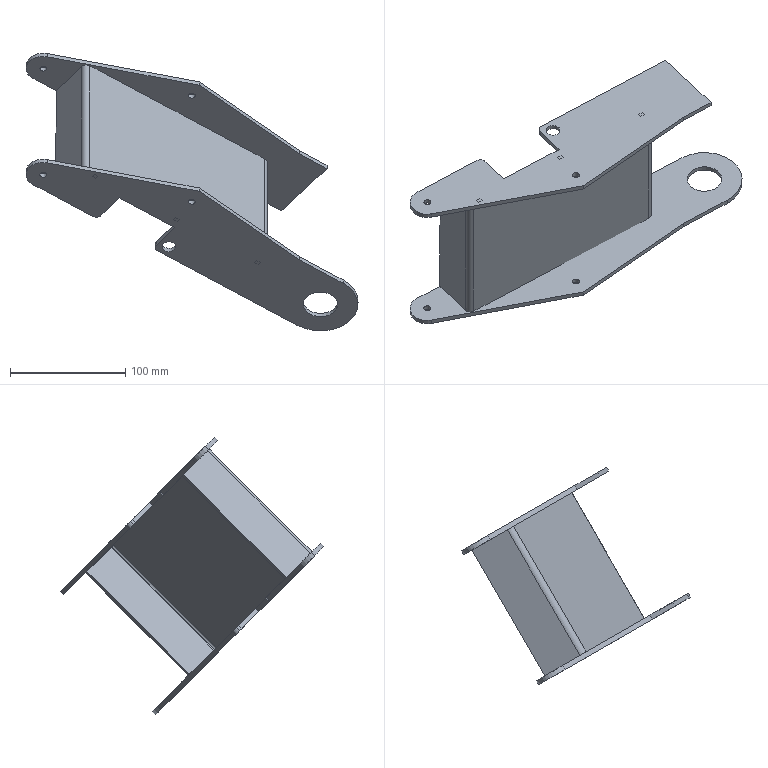Component | SolidWorks | SmallAxisAssembly-1_VegetablePressSide-1 | 3 solids | 118 faces | volume 236923 mm3 | plane 87 | cylinder 31 | commonest cylinder face diameters 10 x9 6 x8 30 x6 12 x4 4 x3 65 x1